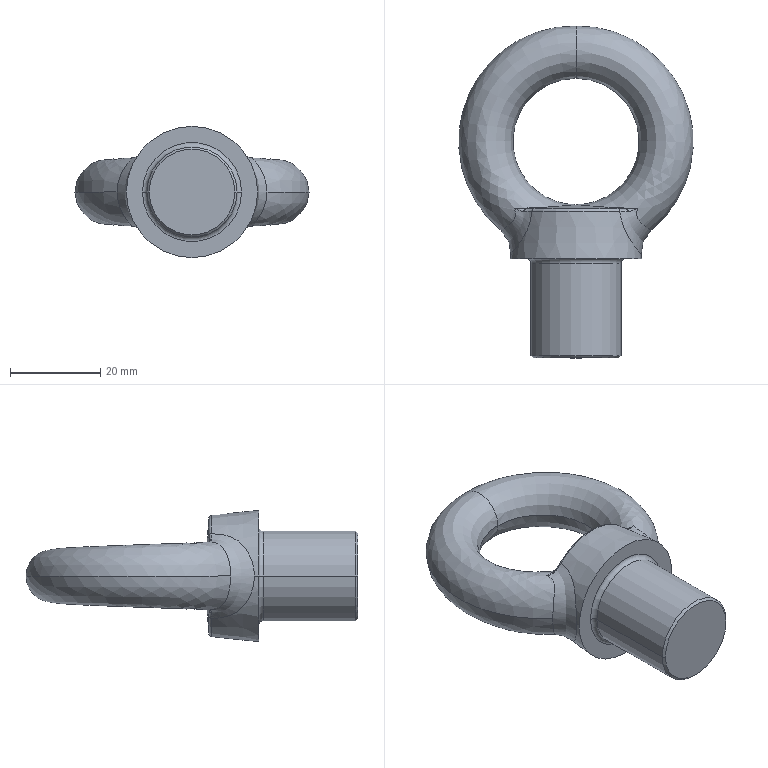Component | SolidWorks | GB_T825-1988[LiftingEyeBoltM20]-1 | 1 solid | 32 faces | volume 26355 mm3 | spline 18 | cone 6 | torus 4 | cylinder 2 | plane 2 | commonest cylinder face diameters 20 x2